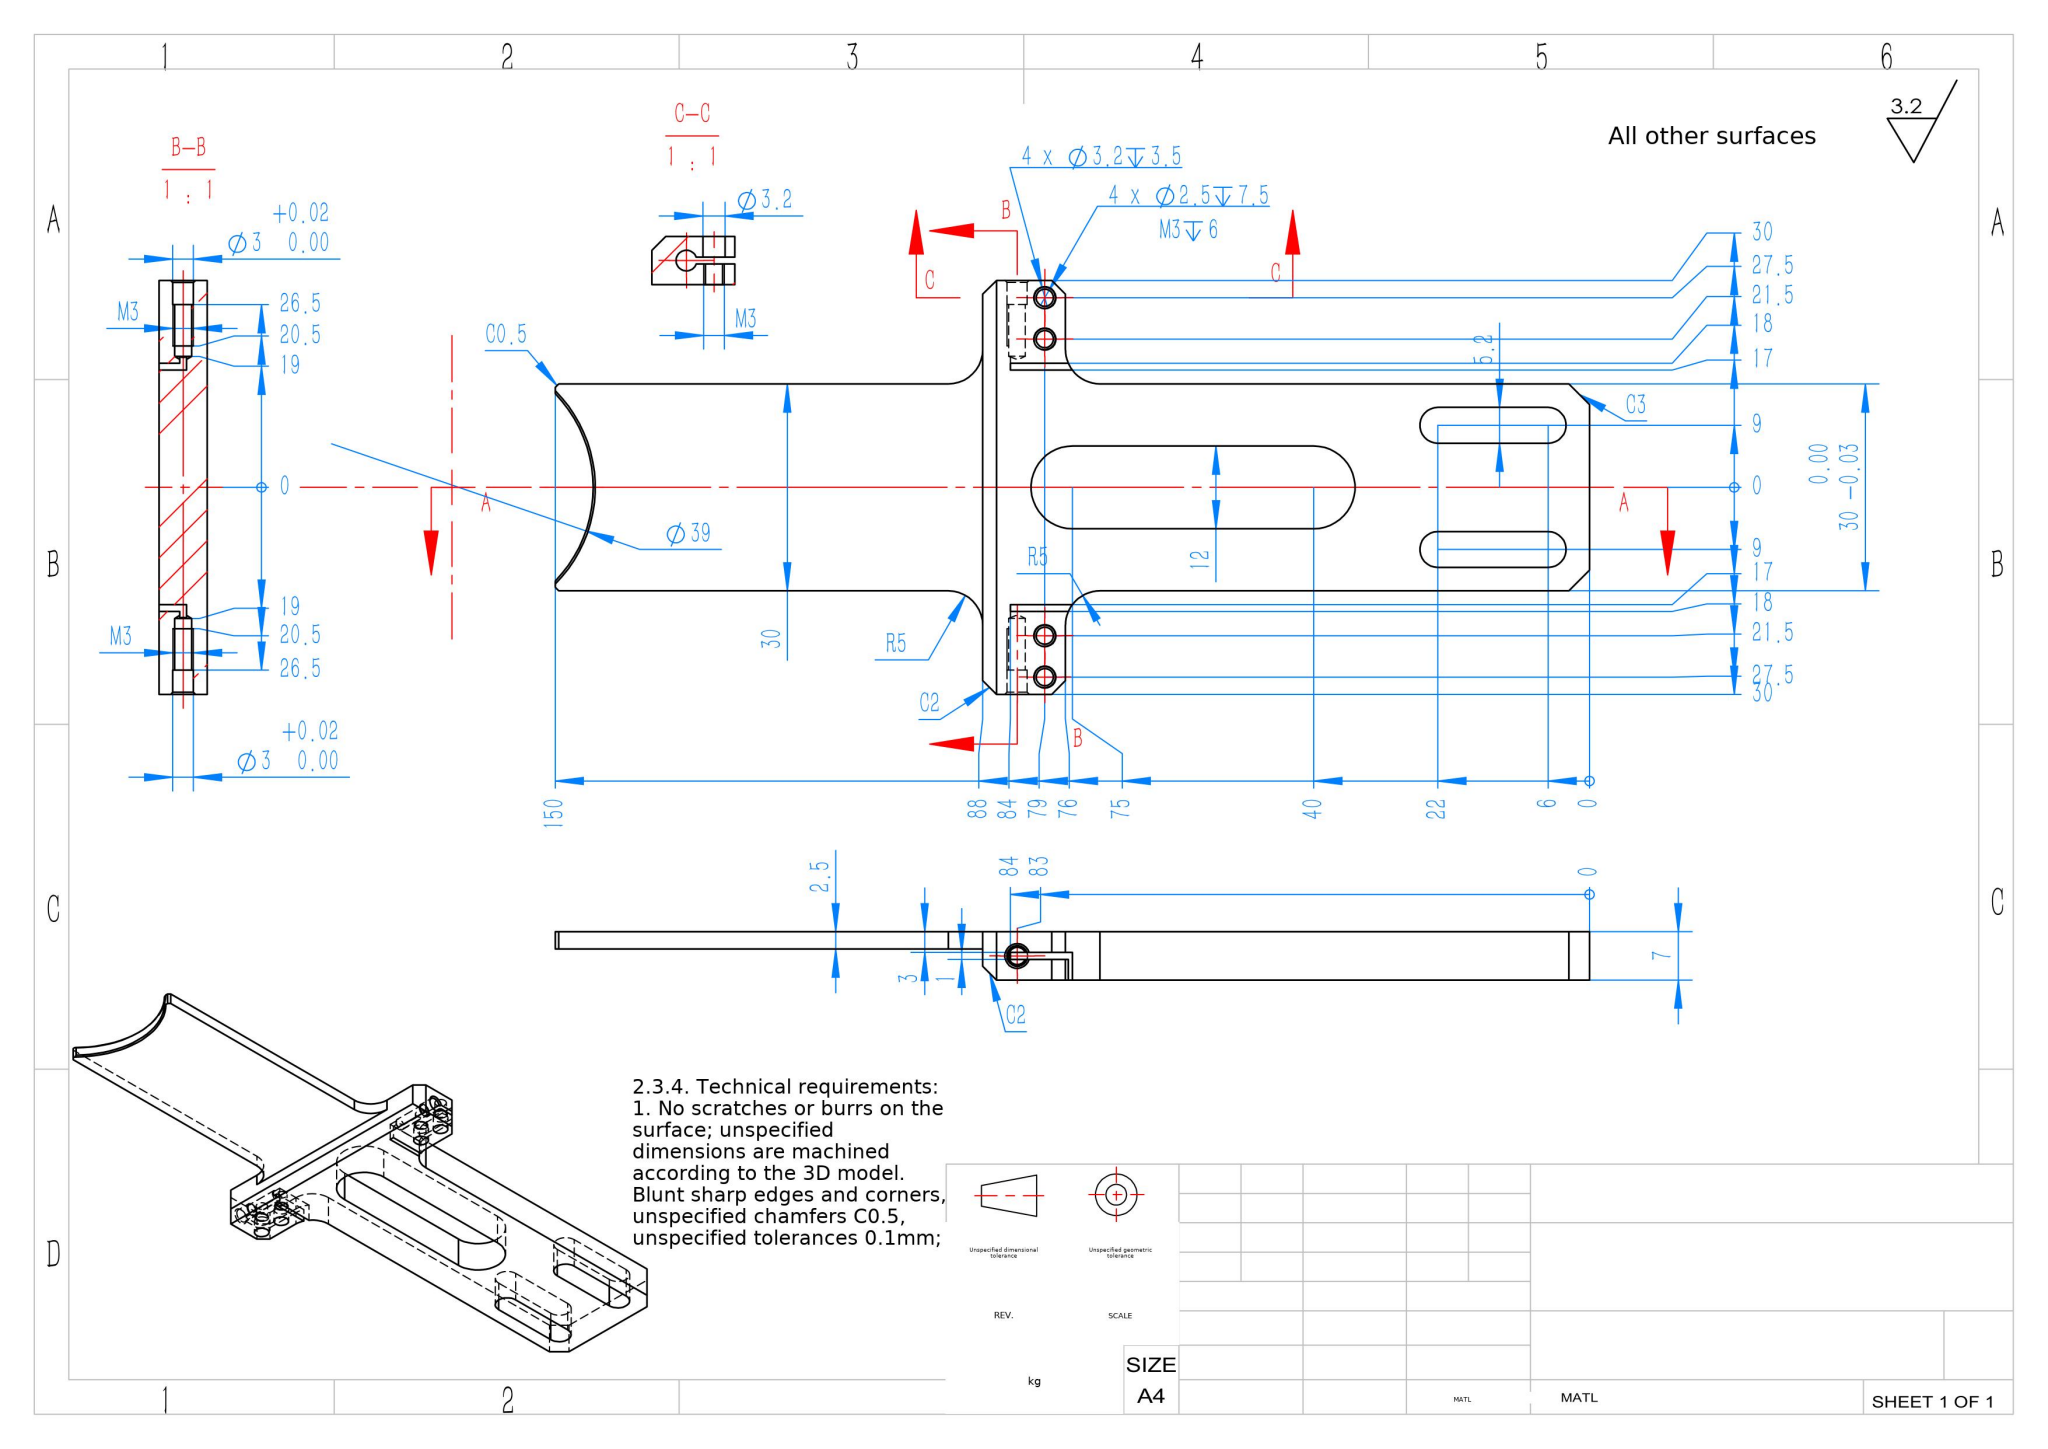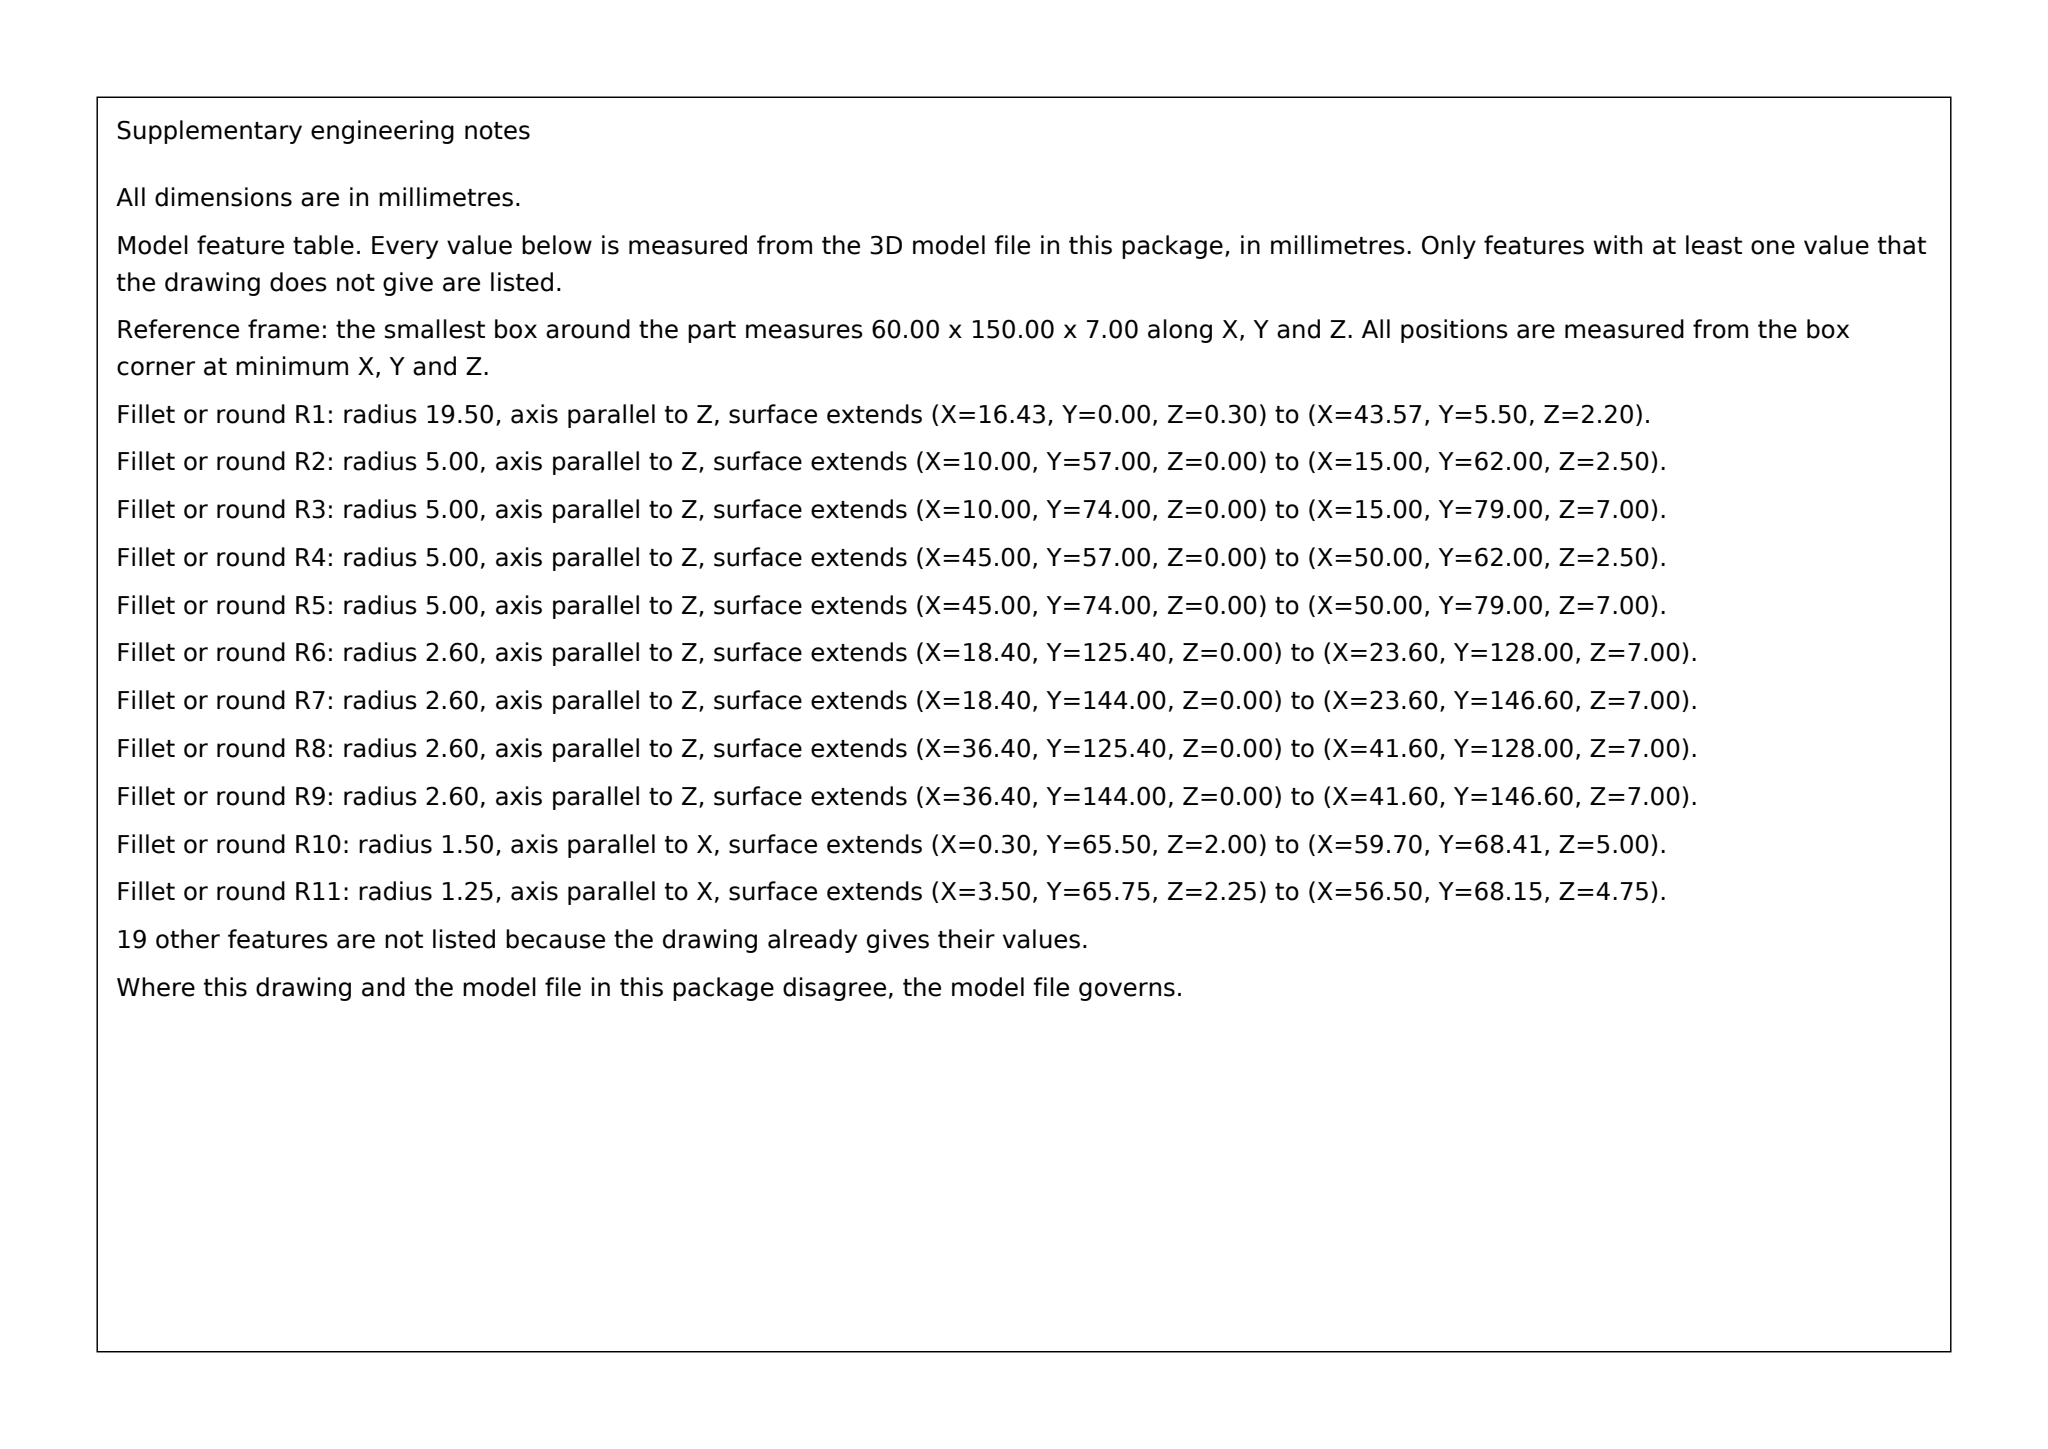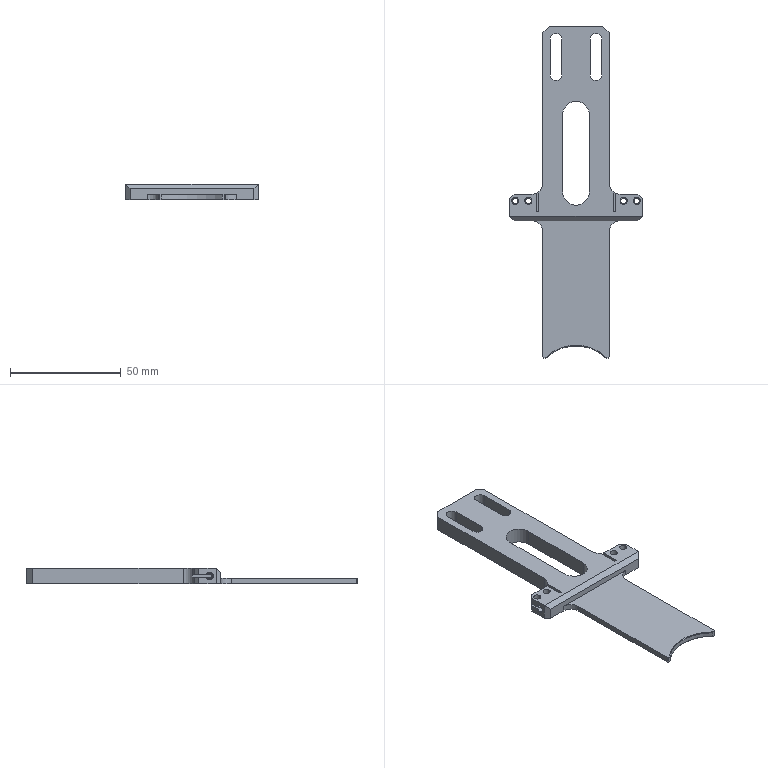Part | SolidWorks | mm | 1 solid | 101 faces | box 60 x 150 x 7 mm | volume 19577 mm3 | plane 46 | cylinder 41 | cone 14 | commonest cylinder face diameters 2.5 x14 3.2 x8 3 x6 10 x6 5.2 x4 12 x2 39 x1